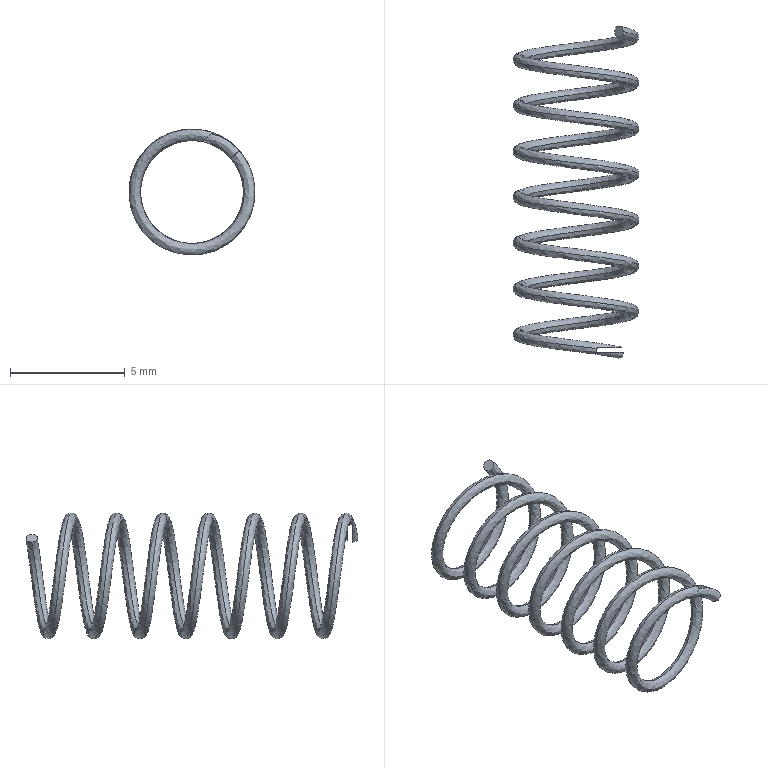Component | SolidWorks | 18Spring1.0-15-1 | 1 solid | 8 faces | box 5.5 x 14.5 x 5.5 mm | volume 21 mm3 | plane 6 | spline 2 | material SKD11